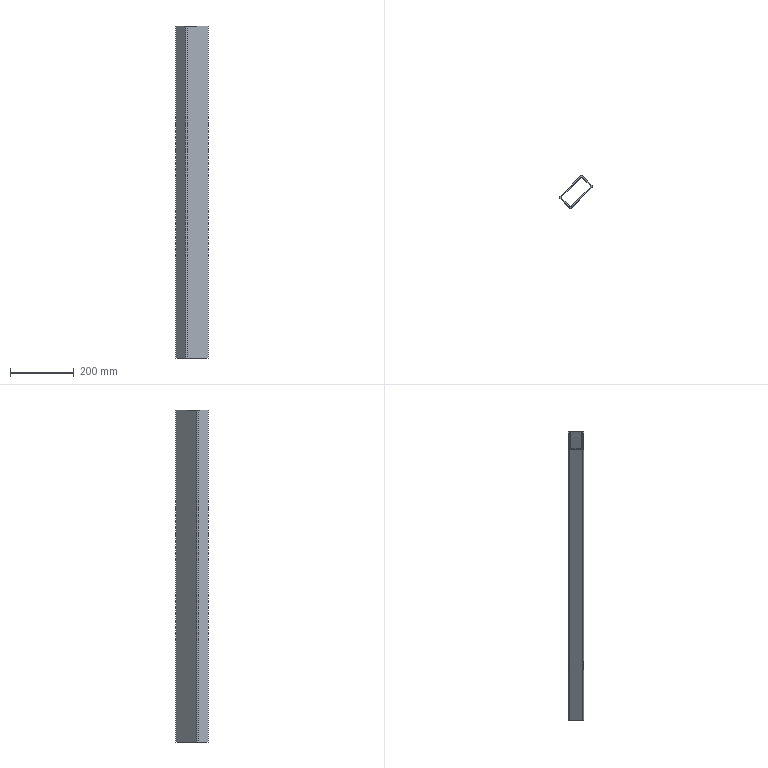Component | NX | CONN_FRAME_CROSS_BEAM | 1 solid | 18 faces | volume 1181440 mm3 | plane 10 | cylinder 8 | commonest cylinder face diameters 8 x8